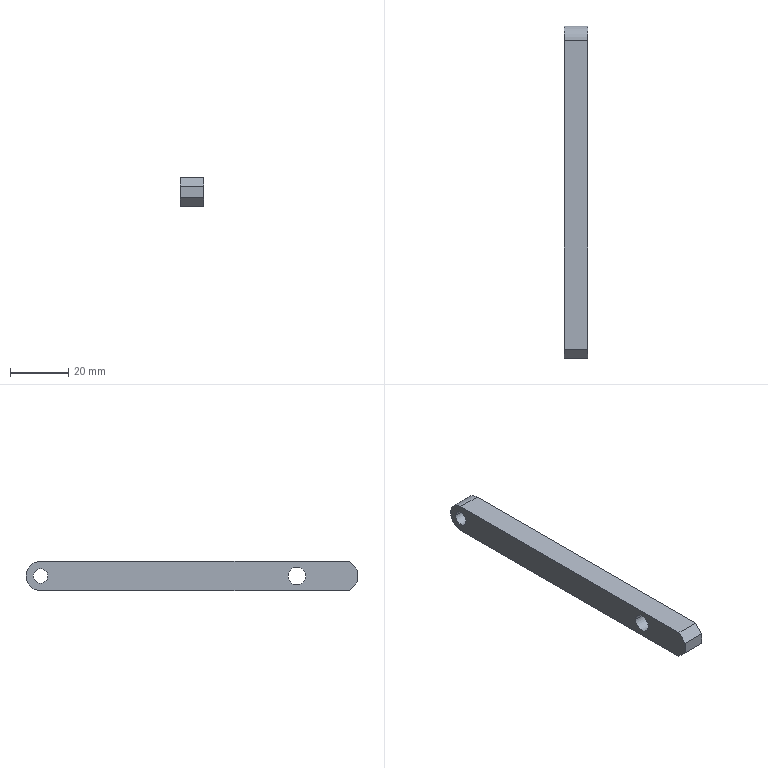Component | SolidWorks | A48-1 | 1 solid | 13 faces | box 8 x 114 x 10 mm | volume 8579 mm3 | plane 7 | cylinder 6 | commonest cylinder face diameters 5 x2 6 x2 10 x2 | material S136
STEP:
#1=COLOUR_RGB('',0.7922,0.8196,0.9333);
#2=FILL_AREA_STYLE_COLOUR('',#1);
#3=FILL_AREA_STYLE('',(#2));
#4=SURFACE_STYLE_FILL_AREA(#3);
#5=SURFACE_SIDE_STYLE('',(#4));
#6=SURFACE_STYLE_USAGE(.BOTH.,#5);
#7=PRESENTATION_STYLE_ASSIGNMENT((#6));
#8=CARTESIAN_POINT('',(-0.9981,4.384,0.1969));
#9=VERTEX_POINT('',#8);
#10=CARTESIAN_POINT('',(-0.9981,4.581,0.1969));
#11=VERTEX_POINT('',#10);
#12=CARTESIAN_POINT('',(-0.9981,4.483,0.1969));
#13=DIRECTION('',(1.,-0.,0.));
#14=DIRECTION('',(0.,1.,-0.));
#15=AXIS2_PLACEMENT_3D('',#12,#13,#14);
#16=CIRCLE('',#15,0.09843);
#17=EDGE_CURVE('',#9,#11,#16,.T.);
#18=ORIENTED_EDGE('',*,*,#17,.F.);
#19=CARTESIAN_POINT('',(-0.6831,4.384,0.1969));
#20=VERTEX_POINT('',#19);
#21=CARTESIAN_POINT('',(-0.6831,4.384,0.1969));
#22=DIRECTION('',(1.,-0.,0.));
#23=VECTOR('',#22,39.37);
#24=LINE('',#21,#23);
#25=EDGE_CURVE('',#9,#20,#24,.T.);
#26=ORIENTED_EDGE('',*,*,#25,.T.);
#27=CARTESIAN_POINT('',(-0.6831,4.581,0.1969));
#28=VERTEX_POINT('',#27);
#29=CARTESIAN_POINT('',(-0.6831,4.483,0.1969));
#30=DIRECTION('',(1.,-0.,0.));
#31=DIRECTION('',(0.,1.,-0.));
#32=AXIS2_PLACEMENT_3D('',#29,#30,#31);
#33=CIRCLE('',#32,0.09843);
#34=EDGE_CURVE('',#20,#28,#33,.T.);
#35=ORIENTED_EDGE('',*,*,#34,.T.);
#36=CARTESIAN_POINT('',(-0.6831,4.581,0.1969));
#37=DIRECTION('',(1.,-0.,0.));
#38=VECTOR('',#37,39.37);
#39=LINE('',#36,#38);
#40=EDGE_CURVE('',#11,#28,#39,.T.);
#41=ORIENTED_EDGE('',*,*,#40,.F.);
#42=EDGE_LOOP('',(#18,#26,#35,#41));
#43=FACE_OUTER_BOUND('',#42,.T.);
#44=CARTESIAN_POINT('',(-0.6831,4.483,0.1969));
#45=DIRECTION('',(1.,-0.,0.));
#46=DIRECTION('',(0.,1.,-0.));
#47=AXIS2_PLACEMENT_3D('',#44,#45,#46);
#48=CYLINDRICAL_SURFACE('',#47,0.09843);
#49=ADVANCED_FACE('',(#43),#48,.F.);
#50=CARTESIAN_POINT('',(-0.9981,0.9002,0.1969));
#51=VERTEX_POINT('',#50);
#52=CARTESIAN_POINT('',(-0.9981,1.136,0.1969));
#53=VERTEX_POINT('',#52);
#54=CARTESIAN_POINT('',(-0.9981,1.018,0.1969));
#55=DIRECTION('',(1.,-0.,0.));
#56=DIRECTION('',(0.,1.,-0.));
#57=AXIS2_PLACEMENT_3D('',#54,#55,#56);
#58=CIRCLE('',#57,0.1181);
#59=EDGE_CURVE('',#51,#53,#58,.T.);
#60=ORIENTED_EDGE('',*,*,#59,.F.);
#61=CARTESIAN_POINT('',(-0.6831,0.9002,0.1969));
#62=VERTEX_POINT('',#61);
#63=CARTESIAN_POINT('',(-0.6831,0.9002,0.1969));
#64=DIRECTION('',(1.,-0.,0.));
#65=VECTOR('',#64,39.37);
#66=LINE('',#63,#65);
#67=EDGE_CURVE('',#51,#62,#66,.T.);
#68=ORIENTED_EDGE('',*,*,#67,.T.);
#69=CARTESIAN_POINT('',(-0.6831,1.136,0.1969));
#70=VERTEX_POINT('',#69);
#71=CARTESIAN_POINT('',(-0.6831,1.018,0.1969));
#72=DIRECTION('',(1.,-0.,0.));
#73=DIRECTION('',(0.,1.,-0.));
#74=AXIS2_PLACEMENT_3D('',#71,#72,#73);
#75=CIRCLE('',#74,0.1181);
#76=EDGE_CURVE('',#62,#70,#75,.T.);
#77=ORIENTED_EDGE('',*,*,#76,.T.);
#78=CARTESIAN_POINT('',(-0.6831,1.136,0.1969));
#79=DIRECTION('',(1.,-0.,0.));
#80=VECTOR('',#79,39.37);
#81=LINE('',#78,#80);
#82=EDGE_CURVE('',#53,#70,#81,.T.);
#83=ORIENTED_EDGE('',*,*,#82,.F.);
#84=EDGE_LOOP('',(#60,#68,#77,#83));
#85=FACE_OUTER_BOUND('',#84,.T.);
#86=CARTESIAN_POINT('',(-0.6831,1.018,0.1969));
#87=DIRECTION('',(1.,-0.,0.));
#88=DIRECTION('',(0.,1.,-0.));
#89=AXIS2_PLACEMENT_3D('',#86,#87,#88);
#90=CYLINDRICAL_SURFACE('',#89,0.1181);
#91=ADVANCED_FACE('',(#85),#90,.F.);
#92=CARTESIAN_POINT('',(-0.9981,4.483,0.3937));
#93=VERTEX_POINT('',#92);
#94=CARTESIAN_POINT('',(-0.9981,0.3096,0.3937));
#95=VERTEX_POINT('',#94);
#96=CARTESIAN_POINT('',(-0.9981,0.1915,0.3937));
#97=DIRECTION('',(-0.,-1.,0.));
#98=VECTOR('',#97,39.37);
#99=LINE('',#96,#98);
#100=EDGE_CURVE('',#93,#95,#99,.T.);
#101=ORIENTED_EDGE('',*,*,#100,.T.);
#102=CARTESIAN_POINT('',(-0.6831,0.3096,0.3937));
#103=VERTEX_POINT('',#102);
#104=CARTESIAN_POINT('',(-0.6831,0.3096,0.3937));
#105=DIRECTION('',(1.,-0.,0.));
#106=VECTOR('',#105,39.37);
#107=LINE('',#104,#106);
#108=EDGE_CURVE('',#95,#103,#107,.T.);
#109=ORIENTED_EDGE('',*,*,#108,.T.);
#110=CARTESIAN_POINT('',(-0.6831,4.483,0.3937));
#111=VERTEX_POINT('',#110);
#112=CARTESIAN_POINT('',(-0.6831,0.1915,0.3937));
#113=DIRECTION('',(-0.,-1.,0.));
#114=VECTOR('',#113,39.37);
#115=LINE('',#112,#114);
#116=EDGE_CURVE('',#111,#103,#115,.T.);
#117=ORIENTED_EDGE('',*,*,#116,.F.);
#118=CARTESIAN_POINT('',(-0.6831,4.483,0.3937));
#119=DIRECTION('',(-1.,0.,-0.));
#120=VECTOR('',#119,39.37);
#121=LINE('',#118,#120);
#122=EDGE_CURVE('',#111,#93,#121,.T.);
#123=ORIENTED_EDGE('',*,*,#122,.T.);
#124=EDGE_LOOP('',(#101,#109,#117,#123));
#125=FACE_OUTER_BOUND('',#124,.T.);
#126=CARTESIAN_POINT('',(-0.6831,0.1915,0.3937));
#127=DIRECTION('',(0.,-0.,-1.));
#128=DIRECTION('',(0.,1.,-0.));
#129=AXIS2_PLACEMENT_3D('',#126,#127,#128);
#130=PLANE('',#129);
#131=ADVANCED_FACE('',(#125),#130,.F.);
#132=CARTESIAN_POINT('',(-0.6831,0.1915,0.2756));
#133=VERTEX_POINT('',#132);
#134=CARTESIAN_POINT('',(-0.6831,0.1915,0.1181));
#135=VERTEX_POINT('',#134);
#136=CARTESIAN_POINT('',(-0.6831,0.1915,0.3937));
#137=DIRECTION('',(0.,-0.,-1.));
#138=VECTOR('',#137,39.37);
#139=LINE('',#136,#138);
#140=EDGE_CURVE('',#133,#135,#139,.T.);
#141=ORIENTED_EDGE('',*,*,#140,.F.);
#142=CARTESIAN_POINT('',(-0.9981,0.1915,0.2756));
#143=VERTEX_POINT('',#142);
#144=CARTESIAN_POINT('',(-0.6831,0.1915,0.2756));
#145=DIRECTION('',(-1.,0.,-0.));
#146=VECTOR('',#145,39.37);
#147=LINE('',#144,#146);
#148=EDGE_CURVE('',#133,#143,#147,.T.);
#149=ORIENTED_EDGE('',*,*,#148,.T.);
#150=CARTESIAN_POINT('',(-0.9981,0.1915,0.1181));
#151=VERTEX_POINT('',#150);
#152=CARTESIAN_POINT('',(-0.9981,0.1915,0.3937));
#153=DIRECTION('',(0.,-0.,-1.));
#154=VECTOR('',#153,39.37);
#155=LINE('',#152,#154);
#156=EDGE_CURVE('',#143,#151,#155,.T.);
#157=ORIENTED_EDGE('',*,*,#156,.T.);
#158=CARTESIAN_POINT('',(-0.6831,0.1915,0.1181));
#159=DIRECTION('',(1.,-0.,0.));
#160=VECTOR('',#159,39.37);
#161=LINE('',#158,#160);
#162=EDGE_CURVE('',#151,#135,#161,.T.);
#163=ORIENTED_EDGE('',*,*,#162,.T.);
#164=EDGE_LOOP('',(#141,#149,#157,#163));
#165=FACE_OUTER_BOUND('',#164,.T.);
#166=CARTESIAN_POINT('',(-0.6831,0.1915,0.3937));
#167=DIRECTION('',(0.,1.,-0.));
#168=DIRECTION('',(-1.,0.,-0.));
#169=AXIS2_PLACEMENT_3D('',#166,#167,#168);
#170=PLANE('',#169);
#171=ADVANCED_FACE('',(#165),#170,.F.);
#172=CARTESIAN_POINT('',(-0.6831,0.3096,0.));
#173=VERTEX_POINT('',#172);
#174=CARTESIAN_POINT('',(-0.6831,4.483,-0.));
#175=VERTEX_POINT('',#174);
#176=CARTESIAN_POINT('',(-0.6831,0.1915,0.));
#177=DIRECTION('',(0.,1.,-0.));
#178=VECTOR('',#177,39.37);
#179=LINE('',#176,#178);
#180=EDGE_CURVE('',#173,#175,#179,.T.);
#181=ORIENTED_EDGE('',*,*,#180,.F.);
#182=CARTESIAN_POINT('',(-0.9981,0.3096,0.));
#183=VERTEX_POINT('',#182);
#184=CARTESIAN_POINT('',(-0.6831,0.3096,0.));
#185=DIRECTION('',(-1.,0.,-0.));
#186=VECTOR('',#185,39.37);
#187=LINE('',#184,#186);
#188=EDGE_CURVE('',#173,#183,#187,.T.);
#189=ORIENTED_EDGE('',*,*,#188,.T.);
#190=CARTESIAN_POINT('',(-0.9981,4.483,-0.));
#191=VERTEX_POINT('',#190);
#192=CARTESIAN_POINT('',(-0.9981,0.1915,0.));
#193=DIRECTION('',(0.,1.,-0.));
#194=VECTOR('',#193,39.37);
#195=LINE('',#192,#194);
#196=EDGE_CURVE('',#183,#191,#195,.T.);
#197=ORIENTED_EDGE('',*,*,#196,.T.);
#198=CARTESIAN_POINT('',(-0.6831,4.483,-0.));
#199=DIRECTION('',(1.,-0.,0.));
#200=VECTOR('',#199,39.37);
#201=LINE('',#198,#200);
#202=EDGE_CURVE('',#191,#175,#201,.T.);
#203=ORIENTED_EDGE('',*,*,#202,.T.);
#204=EDGE_LOOP('',(#181,#189,#197,#203));
#205=FACE_OUTER_BOUND('',#204,.T.);
#206=CARTESIAN_POINT('',(-0.6831,0.1915,0.));
#207=DIRECTION('',(-0.,0.,1.));
#208=DIRECTION('',(-0.,-1.,0.));
#209=AXIS2_PLACEMENT_3D('',#206,#207,#208);
#210=PLANE('',#209);
#211=ADVANCED_FACE('',(#205),#210,.F.);
#212=CARTESIAN_POINT('',(-0.6831,4.483,0.1969));
#213=DIRECTION('',(1.,-0.,0.));
#214=DIRECTION('',(0.,1.,-0.));
#215=AXIS2_PLACEMENT_3D('',#212,#213,#214);
#216=CIRCLE('',#215,0.09843);
#217=EDGE_CURVE('',#28,#20,#216,.T.);
#218=ORIENTED_EDGE('',*,*,#217,.F.);
#219=ORIENTED_EDGE('',*,*,#34,.F.);
#220=EDGE_LOOP('',(#218,#219));
#221=FACE_BOUND('',#220,.T.);
#222=CARTESIAN_POINT('',(-0.6831,1.018,0.1969));
#223=DIRECTION('',(1.,-0.,0.));
#224=DIRECTION('',(0.,1.,-0.));
#225=AXIS2_PLACEMENT_3D('',#222,#223,#224);
#226=CIRCLE('',#225,0.1181);
#227=EDGE_CURVE('',#70,#62,#226,.T.);
#228=ORIENTED_EDGE('',*,*,#227,.F.);
#229=ORIENTED_EDGE('',*,*,#76,.F.);
#230=EDGE_LOOP('',(#228,#229));
#231=FACE_BOUND('',#230,.T.);
#232=ORIENTED_EDGE('',*,*,#116,.T.);
#233=CARTESIAN_POINT('',(-0.6831,1.274,1.358));
#234=DIRECTION('',(0.,-0.7071,-0.7071));
#235=VECTOR('',#234,39.37);
#236=LINE('',#233,#235);
#237=EDGE_CURVE('',#103,#133,#236,.T.);
#238=ORIENTED_EDGE('',*,*,#237,.T.);
#239=ORIENTED_EDGE('',*,*,#140,.T.);
#240=CARTESIAN_POINT('',(-0.6831,1.274,-0.9646));
#241=DIRECTION('',(0.,0.7071,-0.7071));
#242=VECTOR('',#241,39.37);
#243=LINE('',#240,#242);
#244=EDGE_CURVE('',#135,#173,#243,.T.);
#245=ORIENTED_EDGE('',*,*,#244,.T.);
#246=ORIENTED_EDGE('',*,*,#180,.T.);
#247=CARTESIAN_POINT('',(-0.6831,4.68,0.1969));
#248=VERTEX_POINT('',#247);
#249=CARTESIAN_POINT('',(-0.6831,4.483,0.1969));
#250=DIRECTION('',(1.,-0.,0.));
#251=DIRECTION('',(0.,1.,-0.));
#252=AXIS2_PLACEMENT_3D('',#249,#250,#251);
#253=CIRCLE('',#252,0.1969);
#254=EDGE_CURVE('',#175,#248,#253,.T.);
#255=ORIENTED_EDGE('',*,*,#254,.T.);
#256=CARTESIAN_POINT('',(-0.6831,4.483,0.1969));
#257=DIRECTION('',(1.,-0.,0.));
#258=DIRECTION('',(0.,1.,-0.));
#259=AXIS2_PLACEMENT_3D('',#256,#257,#258);
#260=CIRCLE('',#259,0.1969);
#261=EDGE_CURVE('',#248,#111,#260,.T.);
#262=ORIENTED_EDGE('',*,*,#261,.T.);
#263=EDGE_LOOP('',(#232,#238,#239,#245,#246,#255,#262));
#264=FACE_OUTER_BOUND('',#263,.T.);
#265=CARTESIAN_POINT('',(-0.6831,2.436,0.1969));
#266=DIRECTION('',(1.,-0.,0.));
#267=DIRECTION('',(0.,1.,-0.));
#268=AXIS2_PLACEMENT_3D('',#265,#266,#267);
#269=PLANE('',#268);
#270=ADVANCED_FACE('',(#221,#231,#264),#269,.T.);
#271=CARTESIAN_POINT('',(-0.9981,4.483,0.1969));
#272=DIRECTION('',(1.,-0.,0.));
#273=DIRECTION('',(0.,1.,-0.));
#274=AXIS2_PLACEMENT_3D('',#271,#272,#273);
#275=CIRCLE('',#274,0.09843);
#276=EDGE_CURVE('',#11,#9,#275,.T.);
#277=ORIENTED_EDGE('',*,*,#276,.T.);
#278=ORIENTED_EDGE('',*,*,#17,.T.);
#279=EDGE_LOOP('',(#277,#278));
#280=FACE_BOUND('',#279,.T.);
#281=CARTESIAN_POINT('',(-0.9981,1.018,0.1969));
#282=DIRECTION('',(1.,-0.,0.));
#283=DIRECTION('',(0.,1.,-0.));
#284=AXIS2_PLACEMENT_3D('',#281,#282,#283);
#285=CIRCLE('',#284,0.1181);
#286=EDGE_CURVE('',#53,#51,#285,.T.);
#287=ORIENTED_EDGE('',*,*,#286,.T.);
#288=ORIENTED_EDGE('',*,*,#59,.T.);
#289=EDGE_LOOP('',(#287,#288));
#290=FACE_BOUND('',#289,.T.);
#291=ORIENTED_EDGE('',*,*,#156,.F.);
#292=CARTESIAN_POINT('',(-0.9981,0.1915,0.2756));
#293=DIRECTION('',(-0.,0.7071,0.7071));
#294=VECTOR('',#293,39.37);
#295=LINE('',#292,#294);
#296=EDGE_CURVE('',#143,#95,#295,.T.);
#297=ORIENTED_EDGE('',*,*,#296,.T.);
#298=ORIENTED_EDGE('',*,*,#100,.F.);
#299=CARTESIAN_POINT('',(-0.9981,4.68,0.1969));
#300=VERTEX_POINT('',#299);
#301=CARTESIAN_POINT('',(-0.9981,4.483,0.1969));
#302=DIRECTION('',(-1.,0.,-0.));
#303=DIRECTION('',(0.,1.,-0.));
#304=AXIS2_PLACEMENT_3D('',#301,#302,#303);
#305=CIRCLE('',#304,0.1969);
#306=EDGE_CURVE('',#93,#300,#305,.T.);
#307=ORIENTED_EDGE('',*,*,#306,.T.);
#308=CARTESIAN_POINT('',(-0.9981,4.483,0.1969));
#309=DIRECTION('',(-1.,0.,-0.));
#310=DIRECTION('',(0.,1.,-0.));
#311=AXIS2_PLACEMENT_3D('',#308,#309,#310);
#312=CIRCLE('',#311,0.1969);
#313=EDGE_CURVE('',#300,#191,#312,.T.);
#314=ORIENTED_EDGE('',*,*,#313,.T.);
#315=ORIENTED_EDGE('',*,*,#196,.F.);
#316=CARTESIAN_POINT('',(-0.9981,0.3096,0.));
#317=DIRECTION('',(-0.,-0.7071,0.7071));
#318=VECTOR('',#317,39.37);
#319=LINE('',#316,#318);
#320=EDGE_CURVE('',#183,#151,#319,.T.);
#321=ORIENTED_EDGE('',*,*,#320,.T.);
#322=EDGE_LOOP('',(#291,#297,#298,#307,#314,#315,#321));
#323=FACE_OUTER_BOUND('',#322,.T.);
#324=CARTESIAN_POINT('',(-0.9981,2.436,0.1969));
#325=DIRECTION('',(1.,-0.,0.));
#326=DIRECTION('',(0.,1.,-0.));
#327=AXIS2_PLACEMENT_3D('',#324,#325,#326);
#328=PLANE('',#327);
#329=ADVANCED_FACE('',(#280,#290,#323),#328,.F.);
#330=ORIENTED_EDGE('',*,*,#67,.F.);
#331=ORIENTED_EDGE('',*,*,#286,.F.);
#332=ORIENTED_EDGE('',*,*,#82,.T.);
#333=ORIENTED_EDGE('',*,*,#227,.T.);
#334=EDGE_LOOP('',(#330,#331,#332,#333));
#335=FACE_OUTER_BOUND('',#334,.T.);
#336=CARTESIAN_POINT('',(-0.6831,1.018,0.1969));
#337=DIRECTION('',(1.,-0.,0.));
#338=DIRECTION('',(0.,1.,-0.));
#339=AXIS2_PLACEMENT_3D('',#336,#337,#338);
#340=CYLINDRICAL_SURFACE('',#339,0.1181);
#341=ADVANCED_FACE('',(#335),#340,.F.);
#342=CARTESIAN_POINT('',(-0.6831,4.68,0.1969));
#343=DIRECTION('',(-1.,0.,-0.));
#344=VECTOR('',#343,39.37);
#345=LINE('',#342,#344);
#346=EDGE_CURVE('',#248,#300,#345,.T.);
#347=ORIENTED_EDGE('',*,*,#346,.F.);
#348=ORIENTED_EDGE('',*,*,#254,.F.);
#349=ORIENTED_EDGE('',*,*,#202,.F.);
#350=ORIENTED_EDGE('',*,*,#313,.F.);
#351=EDGE_LOOP('',(#347,#348,#349,#350));
#352=FACE_OUTER_BOUND('',#351,.T.);
#353=CARTESIAN_POINT('',(-0.6831,4.483,0.1969));
#354=DIRECTION('',(-1.,0.,-0.));
#355=DIRECTION('',(0.,-1.,0.));
#356=AXIS2_PLACEMENT_3D('',#353,#354,#355);
#357=CYLINDRICAL_SURFACE('',#356,0.1969);
#358=ADVANCED_FACE('',(#352),#357,.T.);
#359=ORIENTED_EDGE('',*,*,#261,.F.);
#360=ORIENTED_EDGE('',*,*,#346,.T.);
#361=ORIENTED_EDGE('',*,*,#306,.F.);
#362=ORIENTED_EDGE('',*,*,#122,.F.);
#363=EDGE_LOOP('',(#359,#360,#361,#362));
#364=FACE_OUTER_BOUND('',#363,.T.);
#365=CARTESIAN_POINT('',(-0.6831,4.483,0.1969));
#366=DIRECTION('',(-1.,0.,-0.));
#367=DIRECTION('',(0.,-1.,0.));
#368=AXIS2_PLACEMENT_3D('',#365,#366,#367);
#369=CYLINDRICAL_SURFACE('',#368,0.1969);
#370=ADVANCED_FACE('',(#364),#369,.T.);
#371=ORIENTED_EDGE('',*,*,#25,.F.);
#372=ORIENTED_EDGE('',*,*,#276,.F.);
#373=ORIENTED_EDGE('',*,*,#40,.T.);
#374=ORIENTED_EDGE('',*,*,#217,.T.);
#375=EDGE_LOOP('',(#371,#372,#373,#374));
#376=FACE_OUTER_BOUND('',#375,.T.);
#377=CARTESIAN_POINT('',(-0.6831,4.483,0.1969));
#378=DIRECTION('',(1.,-0.,0.));
#379=DIRECTION('',(0.,1.,-0.));
#380=AXIS2_PLACEMENT_3D('',#377,#378,#379);
#381=CYLINDRICAL_SURFACE('',#380,0.09843);
#382=ADVANCED_FACE('',(#376),#381,.F.);
#383=ORIENTED_EDGE('',*,*,#237,.F.);
#384=ORIENTED_EDGE('',*,*,#108,.F.);
#385=ORIENTED_EDGE('',*,*,#296,.F.);
#386=ORIENTED_EDGE('',*,*,#148,.F.);
#387=EDGE_LOOP('',(#383,#384,#385,#386));
#388=FACE_OUTER_BOUND('',#387,.T.);
#389=CARTESIAN_POINT('',(-0.6831,0.1915,0.2756));
#390=DIRECTION('',(0.,0.7071,-0.7071));
#391=DIRECTION('',(-1.,0.,-0.));
#392=AXIS2_PLACEMENT_3D('',#389,#390,#391);
#393=PLANE('',#392);
#394=ADVANCED_FACE('',(#388),#393,.F.);
#395=ORIENTED_EDGE('',*,*,#244,.F.);
#396=ORIENTED_EDGE('',*,*,#162,.F.);
#397=ORIENTED_EDGE('',*,*,#320,.F.);
#398=ORIENTED_EDGE('',*,*,#188,.F.);
#399=EDGE_LOOP('',(#395,#396,#397,#398));
#400=FACE_OUTER_BOUND('',#399,.T.);
#401=CARTESIAN_POINT('',(-0.6831,0.3096,0.));
#402=DIRECTION('',(-0.,0.7071,0.7071));
#403=DIRECTION('',(-1.,0.,-0.));
#404=AXIS2_PLACEMENT_3D('',#401,#402,#403);
#405=PLANE('',#404);
#406=ADVANCED_FACE('',(#400),#405,.F.);
#407=CLOSED_SHELL('',(#49,#91,#131,#171,#211,#270,#329,#341,#358,#370,#382,#394,#406));
#408=MANIFOLD_SOLID_BREP('',#407);
#409=STYLED_ITEM('',(#7),#408);
#410=(LENGTH_UNIT()NAMED_UNIT(*)SI_UNIT($,.METRE.));
#411=LENGTH_MEASURE_WITH_UNIT(LENGTH_MEASURE(0.0254),#410);
#412=DIMENSIONAL_EXPONENTS(1.,0.,0.,0.,0.,0.,0.);
#413=(CONVERSION_BASED_UNIT('',#411)LENGTH_UNIT()NAMED_UNIT(#412));
#414=UNCERTAINTY_MEASURE_WITH_UNIT(LENGTH_MEASURE(0.00001),#413,'','');
#415=(NAMED_UNIT(*)PLANE_ANGLE_UNIT()SI_UNIT($,.RADIAN.));
#416=(NAMED_UNIT(*)SI_UNIT($,.STERADIAN.)SOLID_ANGLE_UNIT());
#417=(GEOMETRIC_REPRESENTATION_CONTEXT(3)GLOBAL_UNCERTAINTY_ASSIGNED_CONTEXT((#414))GLOBAL_UNIT_ASSIGNED_CONTEXT((#413,#415,#416))REPRESENTATION_CONTEXT('',''));
#418=MECHANICAL_DESIGN_GEOMETRIC_PRESENTATION_REPRESENTATION('',(#409),#417);
#419=CARTESIAN_POINT('',(0.,0.,0.));
#420=DIRECTION('',(0.,0.,1.));
#421=DIRECTION('',(1.,0.,0.));
#422=AXIS2_PLACEMENT_3D('',#419,#420,#421);
#423=(LENGTH_UNIT()NAMED_UNIT(*)SI_UNIT($,.METRE.));
#424=LENGTH_MEASURE_WITH_UNIT(LENGTH_MEASURE(0.0254),#423);
#425=DIMENSIONAL_EXPONENTS(1.,0.,0.,0.,0.,0.,0.);
#426=(CONVERSION_BASED_UNIT('',#424)LENGTH_UNIT()NAMED_UNIT(#425));
#427=UNCERTAINTY_MEASURE_WITH_UNIT(LENGTH_MEASURE(0.00001),#426,'','');
#428=(NAMED_UNIT(*)PLANE_ANGLE_UNIT()SI_UNIT($,.RADIAN.));
#429=(NAMED_UNIT(*)SI_UNIT($,.STERADIAN.)SOLID_ANGLE_UNIT());
#430=(GEOMETRIC_REPRESENTATION_CONTEXT(3)GLOBAL_UNCERTAINTY_ASSIGNED_CONTEXT((#427))GLOBAL_UNIT_ASSIGNED_CONTEXT((#426,#428,#429))REPRESENTATION_CONTEXT('',''));
#431=ADVANCED_BREP_SHAPE_REPRESENTATION('',(#408,#422),#430);
#432=PRESENTATION_LAYER_ASSIGNMENT('','',(#409));